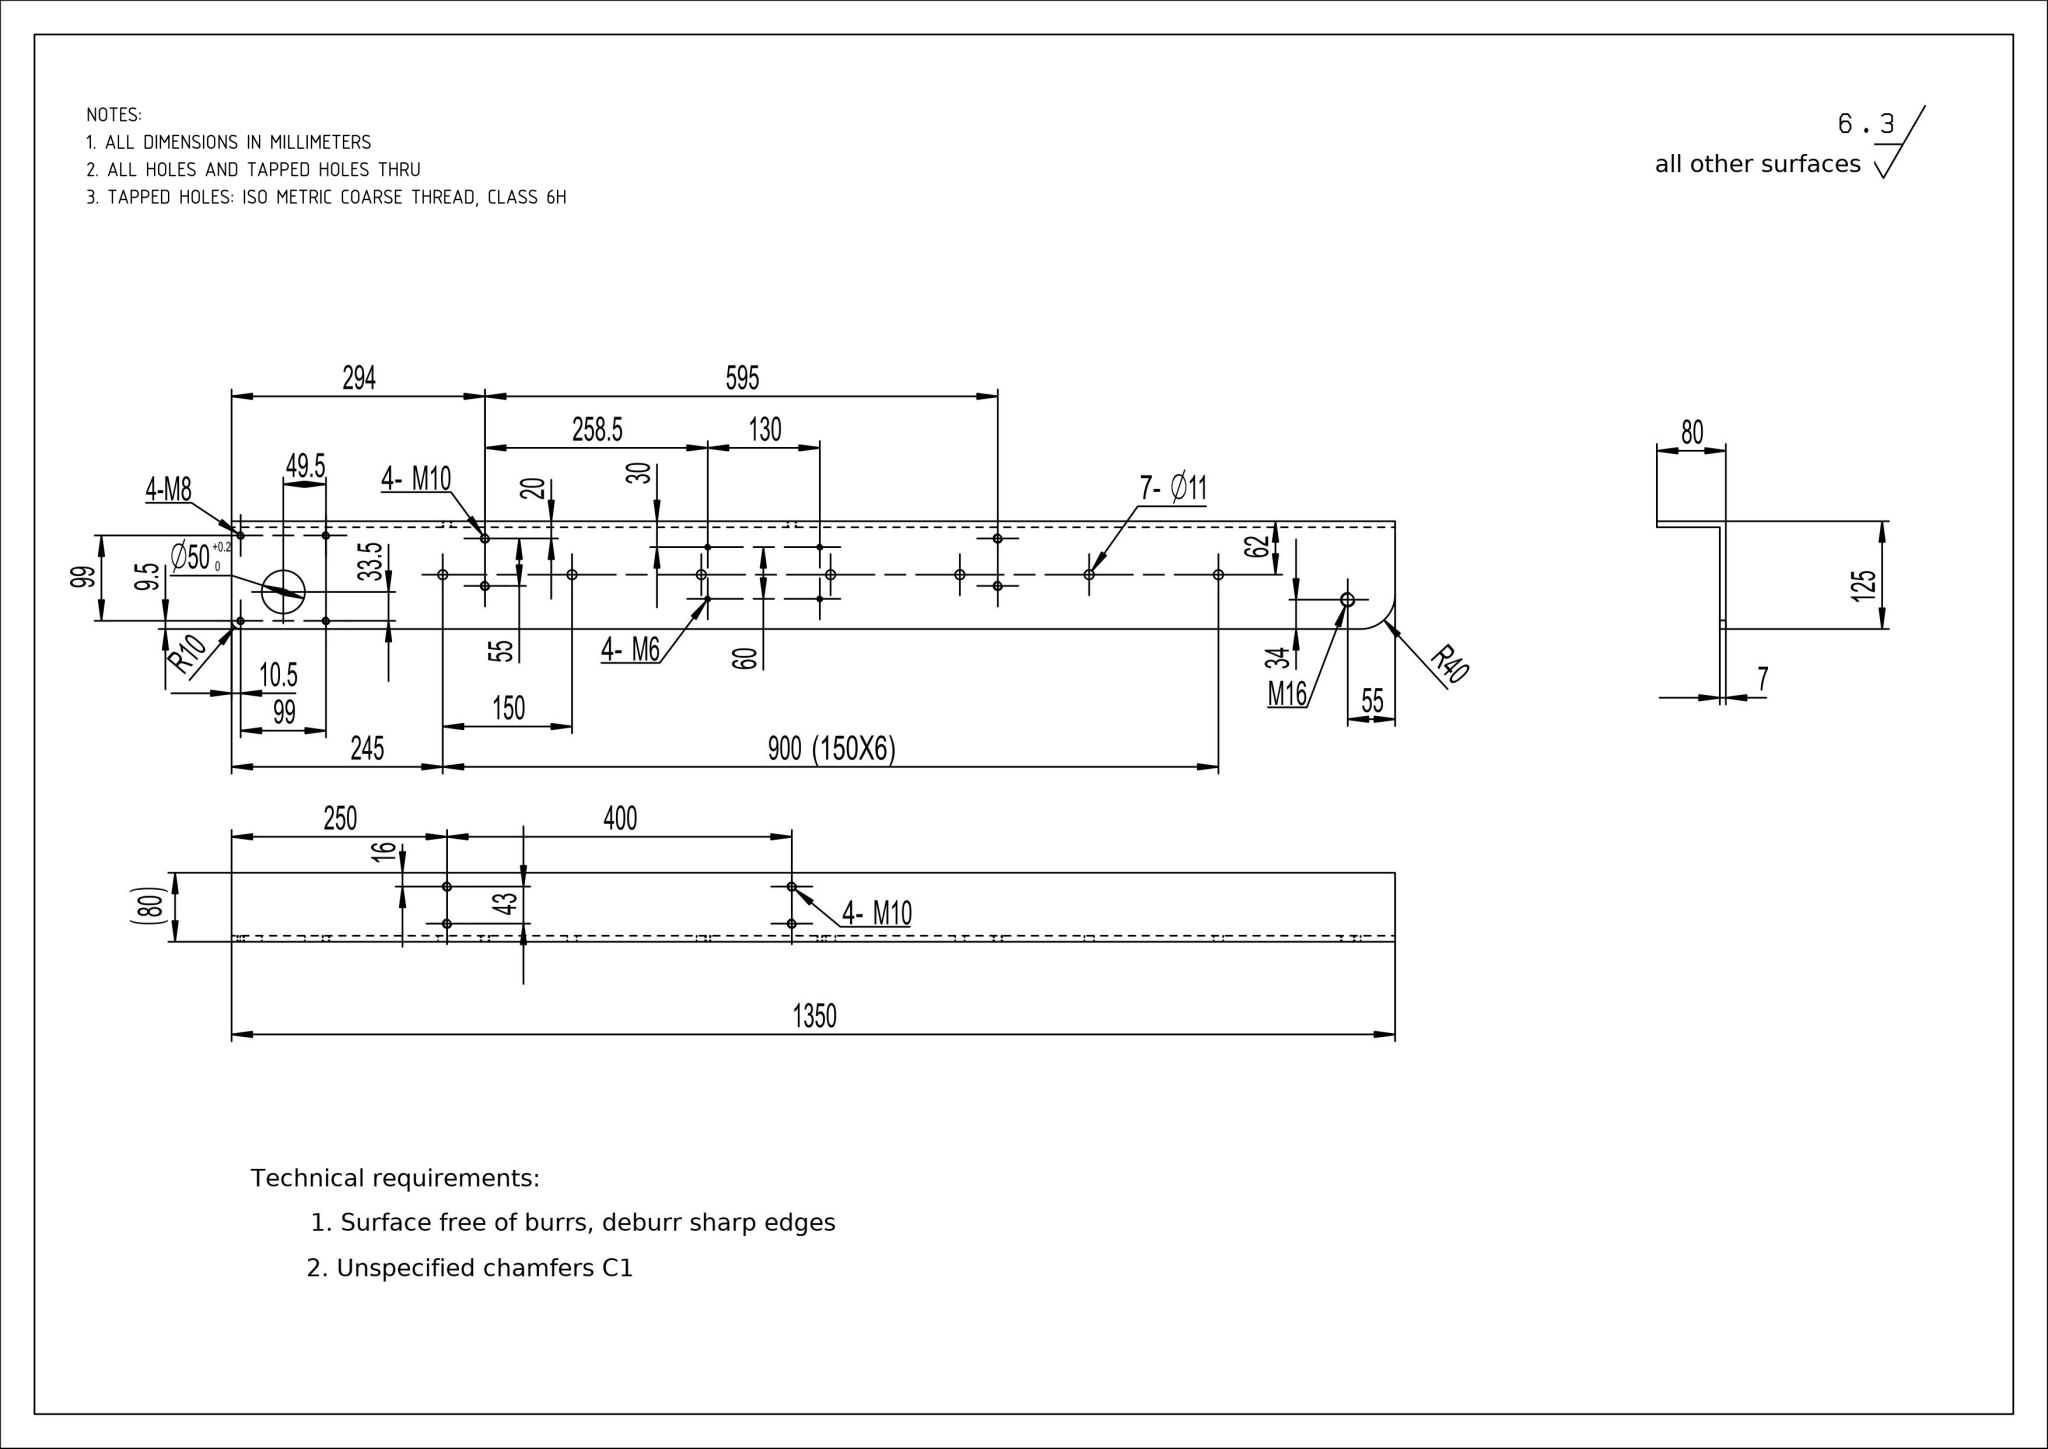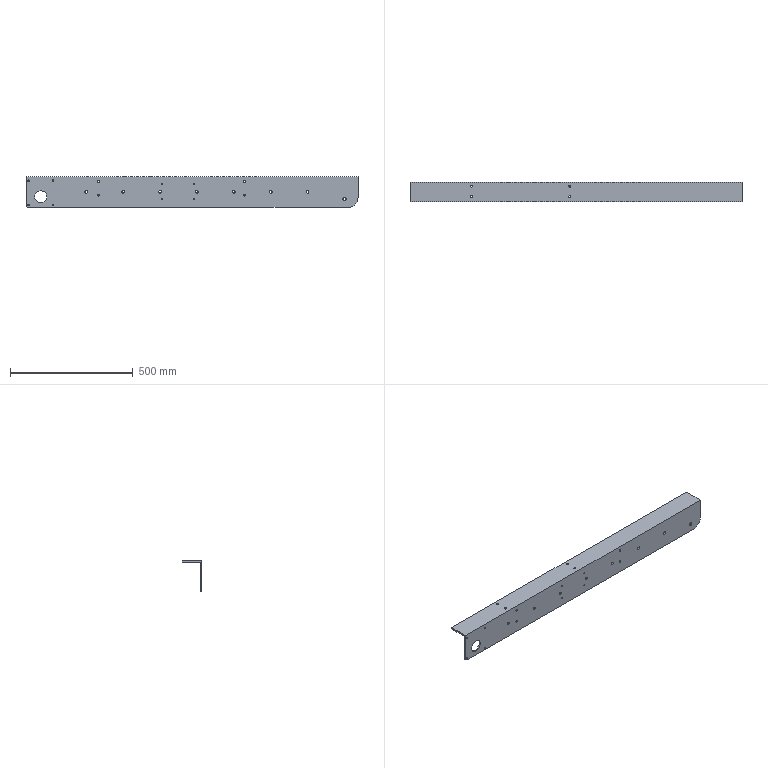Part | NX | mm | 1 solid | 35 faces | box 1350 x 80 x 125 mm | volume 1844353 mm3 | cylinder 27 | plane 8 | commonest cylinder face diameters 8.5 x8 11 x7 5 x4 6.7 x4 50 x1 14 x1 80 x1 20 x1